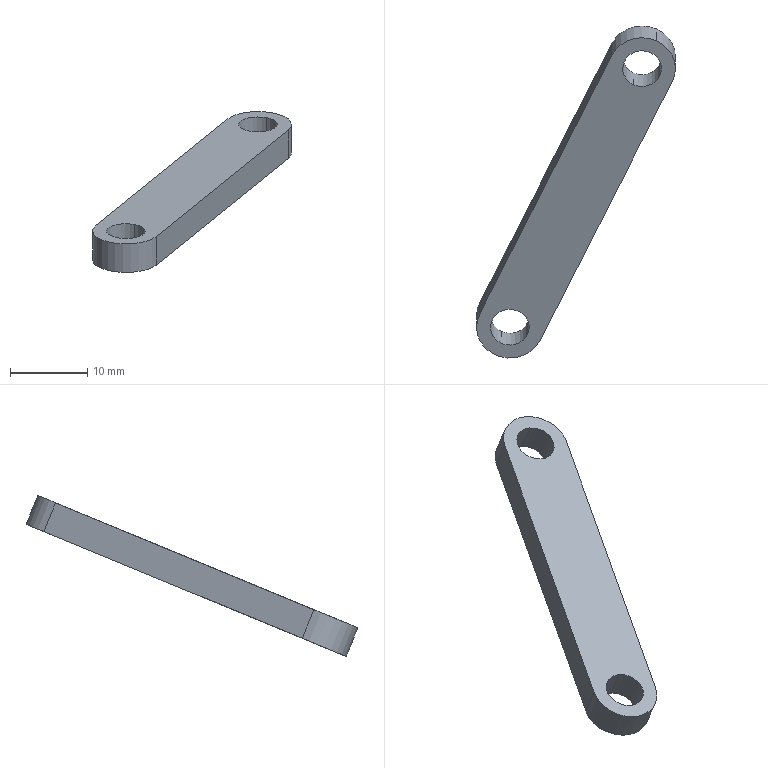Component | SolidWorks | ConnectingRod-1 | 1 solid | 11 faces | box 25.73 x 42.93 x 20.8 mm | volume 1459 mm3 | cylinder 7 | plane 4 | commonest cylinder face diameters 5 x4 8.636 x3
build123d program:
from build123d import *

# Parameters (mm, degrees)
SKETCH1_R           = 2.5
BOSS_EXTRUDE1_DEPTH = 2


with BuildPart() as part:
    # Sketch1 → Boss-Extrude1 (new, symmetric)
    with BuildSketch(Plane.XY):
        with BuildLine():
            Line((0, 4.318), (40, 4.318))
            ThreePointArc((40, 4.318), (44.318, 0), (40, -4.318))
            Line((40, -4.318), (0, -4.318))
            ThreePointArc((0, -4.318), (-4.318, 0), (0, 4.318))
        make_face()
        Circle(SKETCH1_R, mode=Mode.SUBTRACT)
        with Locations((40, 0)):
            Circle(SKETCH1_R, mode=Mode.SUBTRACT)
    extrude(amount=BOSS_EXTRUDE1_DEPTH, both=True)


solid = part.part

# Placed as in the assembly
solid = solid.moved(Location((338.214, 45.724, 9.929), (22.448, 0, -115.294)))
STEP:
#1=COLOUR_RGB('',0.7922,0.8196,0.9333);
#2=FILL_AREA_STYLE_COLOUR('',#1);
#3=FILL_AREA_STYLE('',(#2));
#4=SURFACE_STYLE_FILL_AREA(#3);
#5=SURFACE_SIDE_STYLE('',(#4));
#6=SURFACE_STYLE_USAGE(.BOTH.,#5);
#7=PRESENTATION_STYLE_ASSIGNMENT((#6));
#8=CARTESIAN_POINT('',(12.685,0.5966,-0.1916));
#9=VERTEX_POINT('',#8);
#10=CARTESIAN_POINT('',(12.601,0.4321,-0.2595));
#11=VERTEX_POINT('',#10);
#12=CARTESIAN_POINT('',(12.643,0.5143,-0.2256));
#13=DIRECTION('',(-0.,0.3818,-0.9242));
#14=DIRECTION('',(-0.4273,-0.8356,-0.3452));
#15=AXIS2_PLACEMENT_3D('',#12,#13,#14);
#16=CIRCLE('',#15,0.09843);
#17=EDGE_CURVE('',#9,#11,#16,.T.);
#18=ORIENTED_EDGE('',*,*,#17,.T.);
#19=CARTESIAN_POINT('',(12.601,0.3719,-0.114));
#20=VERTEX_POINT('',#19);
#21=CARTESIAN_POINT('',(12.601,0.4321,-0.2595));
#22=DIRECTION('',(0.,-0.3818,0.9242));
#23=VECTOR('',#22,39.37);
#24=LINE('',#21,#23);
#25=EDGE_CURVE('',#11,#20,#24,.T.);
#26=ORIENTED_EDGE('',*,*,#25,.T.);
#27=CARTESIAN_POINT('',(12.685,0.5364,-0.04603));
#28=VERTEX_POINT('',#27);
#29=CARTESIAN_POINT('',(12.643,0.4542,-0.08002));
#30=DIRECTION('',(-0.,0.3818,-0.9242));
#31=DIRECTION('',(-0.4273,-0.8356,-0.3452));
#32=AXIS2_PLACEMENT_3D('',#29,#30,#31);
#33=CIRCLE('',#32,0.09843);
#34=EDGE_CURVE('',#28,#20,#33,.T.);
#35=ORIENTED_EDGE('',*,*,#34,.F.);
#36=CARTESIAN_POINT('',(12.685,0.5966,-0.1916));
#37=DIRECTION('',(0.,-0.3818,0.9242));
#38=VECTOR('',#37,39.37);
#39=LINE('',#36,#38);
#40=EDGE_CURVE('',#9,#28,#39,.T.);
#41=ORIENTED_EDGE('',*,*,#40,.F.);
#42=EDGE_LOOP('',(#18,#26,#35,#41));
#43=FACE_OUTER_BOUND('',#42,.T.);
#44=CARTESIAN_POINT('',(12.643,0.5143,-0.2256));
#45=DIRECTION('',(0.,-0.3818,0.9242));
#46=DIRECTION('',(0.4273,0.8356,0.3452));
#47=AXIS2_PLACEMENT_3D('',#44,#45,#46);
#48=CYLINDRICAL_SURFACE('',#47,0.09843);
#49=ADVANCED_FACE('',(#43),#48,.F.);
#50=CARTESIAN_POINT('',(13.358,1.912,0.3521));
#51=VERTEX_POINT('',#50);
#52=CARTESIAN_POINT('',(13.273,1.748,0.2841));
#53=VERTEX_POINT('',#52);
#54=CARTESIAN_POINT('',(13.316,1.83,0.3181));
#55=DIRECTION('',(-0.,0.3818,-0.9242));
#56=DIRECTION('',(-0.4273,-0.8356,-0.3452));
#57=AXIS2_PLACEMENT_3D('',#54,#55,#56);
#58=CIRCLE('',#57,0.09843);
#59=EDGE_CURVE('',#51,#53,#58,.T.);
#60=ORIENTED_EDGE('',*,*,#59,.T.);
#61=CARTESIAN_POINT('',(13.273,1.688,0.4297));
#62=VERTEX_POINT('',#61);
#63=CARTESIAN_POINT('',(13.273,1.748,0.2841));
#64=DIRECTION('',(0.,-0.3818,0.9242));
#65=VECTOR('',#64,39.37);
#66=LINE('',#63,#65);
#67=EDGE_CURVE('',#53,#62,#66,.T.);
#68=ORIENTED_EDGE('',*,*,#67,.T.);
#69=CARTESIAN_POINT('',(13.358,1.852,0.4977));
#70=VERTEX_POINT('',#69);
#71=CARTESIAN_POINT('',(13.316,1.77,0.4637));
#72=DIRECTION('',(-0.,0.3818,-0.9242));
#73=DIRECTION('',(-0.4273,-0.8356,-0.3452));
#74=AXIS2_PLACEMENT_3D('',#71,#72,#73);
#75=CIRCLE('',#74,0.09843);
#76=EDGE_CURVE('',#70,#62,#75,.T.);
#77=ORIENTED_EDGE('',*,*,#76,.F.);
#78=CARTESIAN_POINT('',(13.358,1.912,0.3521));
#79=DIRECTION('',(0.,-0.3818,0.9242));
#80=VECTOR('',#79,39.37);
#81=LINE('',#78,#80);
#82=EDGE_CURVE('',#51,#70,#81,.T.);
#83=ORIENTED_EDGE('',*,*,#82,.F.);
#84=EDGE_LOOP('',(#60,#68,#77,#83));
#85=FACE_OUTER_BOUND('',#84,.T.);
#86=CARTESIAN_POINT('',(13.316,1.83,0.3181));
#87=DIRECTION('',(0.,-0.3818,0.9242));
#88=DIRECTION('',(0.4273,0.8356,0.3452));
#89=AXIS2_PLACEMENT_3D('',#86,#87,#88);
#90=CYLINDRICAL_SURFACE('',#89,0.09843);
#91=ADVANCED_FACE('',(#85),#90,.F.);
#92=CARTESIAN_POINT('',(13.388,1.972,0.3768));
#93=VERTEX_POINT('',#92);
#94=CARTESIAN_POINT('',(13.469,1.763,0.2904));
#95=VERTEX_POINT('',#94);
#96=CARTESIAN_POINT('',(13.316,1.83,0.3181));
#97=DIRECTION('',(-0.,0.3818,-0.9242));
#98=DIRECTION('',(-0.4273,-0.8356,-0.3452));
#99=AXIS2_PLACEMENT_3D('',#96,#97,#98);
#100=CIRCLE('',#99,0.17);
#101=EDGE_CURVE('',#93,#95,#100,.T.);
#102=ORIENTED_EDGE('',*,*,#101,.F.);
#103=CARTESIAN_POINT('',(13.388,1.912,0.5224));
#104=VERTEX_POINT('',#103);
#105=CARTESIAN_POINT('',(13.388,1.972,0.3768));
#106=DIRECTION('',(0.,-0.3818,0.9242));
#107=VECTOR('',#106,39.37);
#108=LINE('',#105,#107);
#109=EDGE_CURVE('',#93,#104,#108,.T.);
#110=ORIENTED_EDGE('',*,*,#109,.T.);
#111=CARTESIAN_POINT('',(13.469,1.703,0.4359));
#112=VERTEX_POINT('',#111);
#113=CARTESIAN_POINT('',(13.316,1.77,0.4637));
#114=DIRECTION('',(-0.,0.3818,-0.9242));
#115=DIRECTION('',(-0.4273,-0.8356,-0.3452));
#116=AXIS2_PLACEMENT_3D('',#113,#114,#115);
#117=CIRCLE('',#116,0.17);
#118=EDGE_CURVE('',#104,#112,#117,.T.);
#119=ORIENTED_EDGE('',*,*,#118,.T.);
#120=CARTESIAN_POINT('',(13.469,1.763,0.2904));
#121=DIRECTION('',(0.,-0.3818,0.9242));
#122=VECTOR('',#121,39.37);
#123=LINE('',#120,#122);
#124=EDGE_CURVE('',#95,#112,#123,.T.);
#125=ORIENTED_EDGE('',*,*,#124,.F.);
#126=EDGE_LOOP('',(#102,#110,#119,#125));
#127=FACE_OUTER_BOUND('',#126,.T.);
#128=CARTESIAN_POINT('',(13.316,1.83,0.3181));
#129=DIRECTION('',(0.,-0.3818,0.9242));
#130=DIRECTION('',(0.4273,0.8356,0.3452));
#131=AXIS2_PLACEMENT_3D('',#128,#129,#130);
#132=CYLINDRICAL_SURFACE('',#131,0.17);
#133=ADVANCED_FACE('',(#127),#132,.T.);
#134=ORIENTED_EDGE('',*,*,#59,.F.);
#135=CARTESIAN_POINT('',(13.316,1.83,0.3181));
#136=DIRECTION('',(-0.,0.3818,-0.9242));
#137=DIRECTION('',(-0.4273,-0.8356,-0.3452));
#138=AXIS2_PLACEMENT_3D('',#135,#136,#137);
#139=CIRCLE('',#138,0.09843);
#140=EDGE_CURVE('',#53,#51,#139,.T.);
#141=ORIENTED_EDGE('',*,*,#140,.F.);
#142=EDGE_LOOP('',(#134,#141));
#143=FACE_BOUND('',#142,.T.);
#144=CARTESIAN_POINT('',(13.162,1.897,0.3459));
#145=VERTEX_POINT('',#144);
#146=CARTESIAN_POINT('',(13.316,1.83,0.3181));
#147=DIRECTION('',(-0.,0.3818,-0.9242));
#148=DIRECTION('',(-0.4273,-0.8356,-0.3452));
#149=AXIS2_PLACEMENT_3D('',#146,#147,#148);
#150=CIRCLE('',#149,0.17);
#151=EDGE_CURVE('',#145,#93,#150,.T.);
#152=ORIENTED_EDGE('',*,*,#151,.T.);
#153=ORIENTED_EDGE('',*,*,#101,.T.);
#154=CARTESIAN_POINT('',(12.796,0.4472,-0.2533));
#155=VERTEX_POINT('',#154);
#156=CARTESIAN_POINT('',(13.469,1.763,0.2904));
#157=DIRECTION('',(-0.4273,-0.8356,-0.3452));
#158=VECTOR('',#157,39.37);
#159=LINE('',#156,#158);
#160=EDGE_CURVE('',#95,#155,#159,.T.);
#161=ORIENTED_EDGE('',*,*,#160,.T.);
#162=CARTESIAN_POINT('',(12.489,0.5814,-0.1978));
#163=VERTEX_POINT('',#162);
#164=CARTESIAN_POINT('',(12.643,0.5143,-0.2256));
#165=DIRECTION('',(-0.,0.3818,-0.9242));
#166=DIRECTION('',(-0.4273,-0.8356,-0.3452));
#167=AXIS2_PLACEMENT_3D('',#164,#165,#166);
#168=CIRCLE('',#167,0.17);
#169=EDGE_CURVE('',#155,#163,#168,.T.);
#170=ORIENTED_EDGE('',*,*,#169,.T.);
#171=CARTESIAN_POINT('',(13.162,1.897,0.3459));
#172=DIRECTION('',(0.4273,0.8356,0.3452));
#173=VECTOR('',#172,39.37);
#174=LINE('',#171,#173);
#175=EDGE_CURVE('',#163,#145,#174,.T.);
#176=ORIENTED_EDGE('',*,*,#175,.T.);
#177=EDGE_LOOP('',(#152,#153,#161,#170,#176));
#178=FACE_OUTER_BOUND('',#177,.T.);
#179=ORIENTED_EDGE('',*,*,#17,.F.);
#180=CARTESIAN_POINT('',(12.643,0.5143,-0.2256));
#181=DIRECTION('',(-0.,0.3818,-0.9242));
#182=DIRECTION('',(-0.4273,-0.8356,-0.3452));
#183=AXIS2_PLACEMENT_3D('',#180,#181,#182);
#184=CIRCLE('',#183,0.09843);
#185=EDGE_CURVE('',#11,#9,#184,.T.);
#186=ORIENTED_EDGE('',*,*,#185,.F.);
#187=EDGE_LOOP('',(#179,#186));
#188=FACE_BOUND('',#187,.T.);
#189=CARTESIAN_POINT('',(13.316,1.83,0.3181));
#190=DIRECTION('',(-0.,0.3818,-0.9242));
#191=DIRECTION('',(-0.4273,-0.8356,-0.3452));
#192=AXIS2_PLACEMENT_3D('',#189,#190,#191);
#193=PLANE('',#192);
#194=ADVANCED_FACE('',(#143,#178,#188),#193,.T.);
#195=CARTESIAN_POINT('',(13.162,1.837,0.4914));
#196=VERTEX_POINT('',#195);
#197=CARTESIAN_POINT('',(13.316,1.77,0.4637));
#198=DIRECTION('',(-0.,0.3818,-0.9242));
#199=DIRECTION('',(-0.4273,-0.8356,-0.3452));
#200=AXIS2_PLACEMENT_3D('',#197,#198,#199);
#201=CIRCLE('',#200,0.17);
#202=EDGE_CURVE('',#196,#104,#201,.T.);
#203=ORIENTED_EDGE('',*,*,#202,.F.);
#204=CARTESIAN_POINT('',(12.489,0.5213,-0.05228));
#205=VERTEX_POINT('',#204);
#206=CARTESIAN_POINT('',(13.162,1.837,0.4914));
#207=DIRECTION('',(0.4273,0.8356,0.3452));
#208=VECTOR('',#207,39.37);
#209=LINE('',#206,#208);
#210=EDGE_CURVE('',#205,#196,#209,.T.);
#211=ORIENTED_EDGE('',*,*,#210,.F.);
#212=CARTESIAN_POINT('',(12.796,0.387,-0.1078));
#213=VERTEX_POINT('',#212);
#214=CARTESIAN_POINT('',(12.643,0.4542,-0.08002));
#215=DIRECTION('',(-0.,0.3818,-0.9242));
#216=DIRECTION('',(-0.4273,-0.8356,-0.3452));
#217=AXIS2_PLACEMENT_3D('',#214,#215,#216);
#218=CIRCLE('',#217,0.17);
#219=EDGE_CURVE('',#213,#205,#218,.T.);
#220=ORIENTED_EDGE('',*,*,#219,.F.);
#221=CARTESIAN_POINT('',(13.469,1.703,0.4359));
#222=DIRECTION('',(-0.4273,-0.8356,-0.3452));
#223=VECTOR('',#222,39.37);
#224=LINE('',#221,#223);
#225=EDGE_CURVE('',#112,#213,#224,.T.);
#226=ORIENTED_EDGE('',*,*,#225,.F.);
#227=ORIENTED_EDGE('',*,*,#118,.F.);
#228=EDGE_LOOP('',(#203,#211,#220,#226,#227));
#229=FACE_OUTER_BOUND('',#228,.T.);
#230=ORIENTED_EDGE('',*,*,#76,.T.);
#231=CARTESIAN_POINT('',(13.316,1.77,0.4637));
#232=DIRECTION('',(-0.,0.3818,-0.9242));
#233=DIRECTION('',(-0.4273,-0.8356,-0.3452));
#234=AXIS2_PLACEMENT_3D('',#231,#232,#233);
#235=CIRCLE('',#234,0.09843);
#236=EDGE_CURVE('',#62,#70,#235,.T.);
#237=ORIENTED_EDGE('',*,*,#236,.T.);
#238=EDGE_LOOP('',(#230,#237));
#239=FACE_BOUND('',#238,.T.);
#240=ORIENTED_EDGE('',*,*,#34,.T.);
#241=CARTESIAN_POINT('',(12.643,0.4542,-0.08002));
#242=DIRECTION('',(-0.,0.3818,-0.9242));
#243=DIRECTION('',(-0.4273,-0.8356,-0.3452));
#244=AXIS2_PLACEMENT_3D('',#241,#242,#243);
#245=CIRCLE('',#244,0.09843);
#246=EDGE_CURVE('',#20,#28,#245,.T.);
#247=ORIENTED_EDGE('',*,*,#246,.T.);
#248=EDGE_LOOP('',(#240,#247));
#249=FACE_BOUND('',#248,.T.);
#250=CARTESIAN_POINT('',(13.316,1.77,0.4637));
#251=DIRECTION('',(-0.,0.3818,-0.9242));
#252=DIRECTION('',(-0.4273,-0.8356,-0.3452));
#253=AXIS2_PLACEMENT_3D('',#250,#251,#252);
#254=PLANE('',#253);
#255=ADVANCED_FACE('',(#229,#239,#249),#254,.F.);
#256=ORIENTED_EDGE('',*,*,#109,.F.);
#257=ORIENTED_EDGE('',*,*,#151,.F.);
#258=CARTESIAN_POINT('',(13.162,1.897,0.3459));
#259=DIRECTION('',(0.,-0.3818,0.9242));
#260=VECTOR('',#259,39.37);
#261=LINE('',#258,#260);
#262=EDGE_CURVE('',#145,#196,#261,.T.);
#263=ORIENTED_EDGE('',*,*,#262,.T.);
#264=ORIENTED_EDGE('',*,*,#202,.T.);
#265=EDGE_LOOP('',(#256,#257,#263,#264));
#266=FACE_OUTER_BOUND('',#265,.T.);
#267=CARTESIAN_POINT('',(13.316,1.83,0.3181));
#268=DIRECTION('',(0.,-0.3818,0.9242));
#269=DIRECTION('',(0.4273,0.8356,0.3452));
#270=AXIS2_PLACEMENT_3D('',#267,#268,#269);
#271=CYLINDRICAL_SURFACE('',#270,0.17);
#272=ADVANCED_FACE('',(#266),#271,.T.);
#273=ORIENTED_EDGE('',*,*,#225,.T.);
#274=CARTESIAN_POINT('',(12.796,0.4472,-0.2533));
#275=DIRECTION('',(0.,-0.3818,0.9242));
#276=VECTOR('',#275,39.37);
#277=LINE('',#274,#276);
#278=EDGE_CURVE('',#155,#213,#277,.T.);
#279=ORIENTED_EDGE('',*,*,#278,.F.);
#280=ORIENTED_EDGE('',*,*,#160,.F.);
#281=ORIENTED_EDGE('',*,*,#124,.T.);
#282=EDGE_LOOP('',(#273,#279,#280,#281));
#283=FACE_OUTER_BOUND('',#282,.T.);
#284=CARTESIAN_POINT('',(13.469,1.763,0.2904));
#285=DIRECTION('',(-0.9041,0.3949,0.1631));
#286=DIRECTION('',(-0.,0.3818,-0.9242));
#287=AXIS2_PLACEMENT_3D('',#284,#285,#286);
#288=PLANE('',#287);
#289=ADVANCED_FACE('',(#283),#288,.F.);
#290=ORIENTED_EDGE('',*,*,#219,.T.);
#291=CARTESIAN_POINT('',(12.489,0.5814,-0.1978));
#292=DIRECTION('',(0.,-0.3818,0.9242));
#293=VECTOR('',#292,39.37);
#294=LINE('',#291,#293);
#295=EDGE_CURVE('',#163,#205,#294,.T.);
#296=ORIENTED_EDGE('',*,*,#295,.F.);
#297=ORIENTED_EDGE('',*,*,#169,.F.);
#298=ORIENTED_EDGE('',*,*,#278,.T.);
#299=EDGE_LOOP('',(#290,#296,#297,#298));
#300=FACE_OUTER_BOUND('',#299,.T.);
#301=CARTESIAN_POINT('',(12.643,0.5143,-0.2256));
#302=DIRECTION('',(0.,-0.3818,0.9242));
#303=DIRECTION('',(0.4273,0.8356,0.3452));
#304=AXIS2_PLACEMENT_3D('',#301,#302,#303);
#305=CYLINDRICAL_SURFACE('',#304,0.17);
#306=ADVANCED_FACE('',(#300),#305,.T.);
#307=ORIENTED_EDGE('',*,*,#210,.T.);
#308=ORIENTED_EDGE('',*,*,#262,.F.);
#309=ORIENTED_EDGE('',*,*,#175,.F.);
#310=ORIENTED_EDGE('',*,*,#295,.T.);
#311=EDGE_LOOP('',(#307,#308,#309,#310));
#312=FACE_OUTER_BOUND('',#311,.T.);
#313=CARTESIAN_POINT('',(13.162,1.897,0.3459));
#314=DIRECTION('',(0.9041,-0.3949,-0.1631));
#315=DIRECTION('',(0.,-0.3818,0.9242));
#316=AXIS2_PLACEMENT_3D('',#313,#314,#315);
#317=PLANE('',#316);
#318=ADVANCED_FACE('',(#312),#317,.F.);
#319=ORIENTED_EDGE('',*,*,#67,.F.);
#320=ORIENTED_EDGE('',*,*,#140,.T.);
#321=ORIENTED_EDGE('',*,*,#82,.T.);
#322=ORIENTED_EDGE('',*,*,#236,.F.);
#323=EDGE_LOOP('',(#319,#320,#321,#322));
#324=FACE_OUTER_BOUND('',#323,.T.);
#325=CARTESIAN_POINT('',(13.316,1.83,0.3181));
#326=DIRECTION('',(0.,-0.3818,0.9242));
#327=DIRECTION('',(0.4273,0.8356,0.3452));
#328=AXIS2_PLACEMENT_3D('',#325,#326,#327);
#329=CYLINDRICAL_SURFACE('',#328,0.09843);
#330=ADVANCED_FACE('',(#324),#329,.F.);
#331=ORIENTED_EDGE('',*,*,#25,.F.);
#332=ORIENTED_EDGE('',*,*,#185,.T.);
#333=ORIENTED_EDGE('',*,*,#40,.T.);
#334=ORIENTED_EDGE('',*,*,#246,.F.);
#335=EDGE_LOOP('',(#331,#332,#333,#334));
#336=FACE_OUTER_BOUND('',#335,.T.);
#337=CARTESIAN_POINT('',(12.643,0.5143,-0.2256));
#338=DIRECTION('',(0.,-0.3818,0.9242));
#339=DIRECTION('',(0.4273,0.8356,0.3452));
#340=AXIS2_PLACEMENT_3D('',#337,#338,#339);
#341=CYLINDRICAL_SURFACE('',#340,0.09843);
#342=ADVANCED_FACE('',(#336),#341,.F.);
#343=CLOSED_SHELL('',(#49,#91,#133,#194,#255,#272,#289,#306,#318,#330,#342));
#344=MANIFOLD_SOLID_BREP('',#343);
#345=STYLED_ITEM('',(#7),#344);
#346=(LENGTH_UNIT()NAMED_UNIT(*)SI_UNIT($,.METRE.));
#347=LENGTH_MEASURE_WITH_UNIT(LENGTH_MEASURE(0.0254),#346);
#348=DIMENSIONAL_EXPONENTS(1.,0.,0.,0.,0.,0.,0.);
#349=(CONVERSION_BASED_UNIT('',#347)LENGTH_UNIT()NAMED_UNIT(#348));
#350=UNCERTAINTY_MEASURE_WITH_UNIT(LENGTH_MEASURE(0.00001),#349,'','');
#351=(NAMED_UNIT(*)PLANE_ANGLE_UNIT()SI_UNIT($,.RADIAN.));
#352=(NAMED_UNIT(*)SI_UNIT($,.STERADIAN.)SOLID_ANGLE_UNIT());
#353=(GEOMETRIC_REPRESENTATION_CONTEXT(3)GLOBAL_UNCERTAINTY_ASSIGNED_CONTEXT((#350))GLOBAL_UNIT_ASSIGNED_CONTEXT((#349,#351,#352))REPRESENTATION_CONTEXT('',''));
#354=MECHANICAL_DESIGN_GEOMETRIC_PRESENTATION_REPRESENTATION('',(#345),#353);
#355=CARTESIAN_POINT('',(0.,0.,0.));
#356=DIRECTION('',(0.,0.,1.));
#357=DIRECTION('',(1.,0.,0.));
#358=AXIS2_PLACEMENT_3D('',#355,#356,#357);
#359=(LENGTH_UNIT()NAMED_UNIT(*)SI_UNIT($,.METRE.));
#360=LENGTH_MEASURE_WITH_UNIT(LENGTH_MEASURE(0.0254),#359);
#361=DIMENSIONAL_EXPONENTS(1.,0.,0.,0.,0.,0.,0.);
#362=(CONVERSION_BASED_UNIT('',#360)LENGTH_UNIT()NAMED_UNIT(#361));
#363=UNCERTAINTY_MEASURE_WITH_UNIT(LENGTH_MEASURE(0.00001),#362,'','');
#364=(NAMED_UNIT(*)PLANE_ANGLE_UNIT()SI_UNIT($,.RADIAN.));
#365=(NAMED_UNIT(*)SI_UNIT($,.STERADIAN.)SOLID_ANGLE_UNIT());
#366=(GEOMETRIC_REPRESENTATION_CONTEXT(3)GLOBAL_UNCERTAINTY_ASSIGNED_CONTEXT((#363))GLOBAL_UNIT_ASSIGNED_CONTEXT((#362,#364,#365))REPRESENTATION_CONTEXT('',''));
#367=ADVANCED_BREP_SHAPE_REPRESENTATION('',(#344,#358),#366);
#368=PRESENTATION_LAYER_ASSIGNMENT('','',(#345));